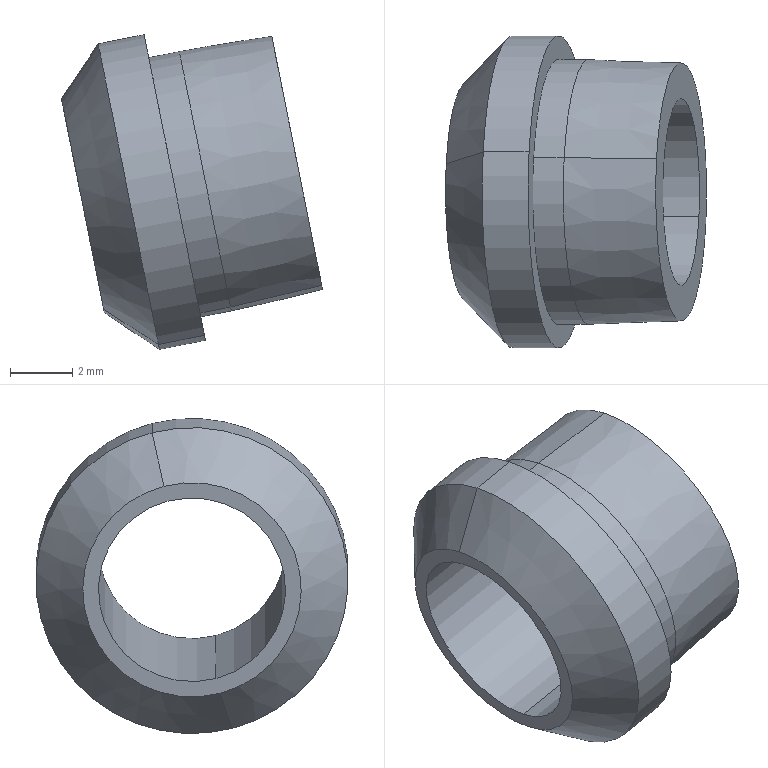Component | SolidWorks | 3-1 | 1 solid | 13 faces | box 8.37 x 10 x 10.1 mm | volume 229 mm3 | cylinder 6 | cone 4 | plane 3 | commonest cylinder face diameters 8.5 x2 10 x2 6 x2
build123d program:
from build123d import *

# Parameters (mm, degrees)
CHAMFER1_SIZE = 1.5


with BuildPart() as part:
    # Sketch1 → Revolve1 (revolve)
    with BuildSketch(Plane(origin=(0, 0, 0), x_dir=(1, 0, 0), z_dir=(0, 1, 0))):
        Polygon((0, 4.145), (3, 4.25), (4, 4.25), (4, 5), (7, 5), (7, 3), (0, 3), align=None)
    revolve(axis=Axis((7, 0, 0), (-1, 0, 0)))

    # Chamfer1
    chamfer1_edges = [part.edges().sort_by_distance(p)[0] for p in [
        (7, 0, 5),
    ]]
    chamfer(chamfer1_edges, length=CHAMFER1_SIZE)


solid = part.part

# Placed as in the assembly
solid = solid.moved(Location((91.677, -319.2, 18.375), (-89.807, -0.03862, 168.666)))
STEP:
#1=COLOUR_RGB('',0.7922,0.8196,0.9333);
#2=FILL_AREA_STYLE_COLOUR('',#1);
#3=FILL_AREA_STYLE('',(#2));
#4=SURFACE_STYLE_FILL_AREA(#3);
#5=SURFACE_SIDE_STYLE('',(#4));
#6=SURFACE_STYLE_USAGE(.BOTH.,#5);
#7=PRESENTATION_STYLE_ASSIGNMENT((#6));
#8=CARTESIAN_POINT('',(3.313,-12.532,0.7999));
#9=VERTEX_POINT('',#8);
#10=CARTESIAN_POINT('',(3.365,-12.602,0.5387));
#11=VERTEX_POINT('',#10);
#12=CARTESIAN_POINT('',(3.339,-12.567,0.6693));
#13=DIRECTION('',(-0.9805,-0.,-0.1965));
#14=DIRECTION('',(-0.19,0.2563,0.9478));
#15=AXIS2_PLACEMENT_3D('',#12,#13,#14);
#16=CIRCLE('',#15,0.1378);
#17=EDGE_CURVE('',#9,#11,#16,.T.);
#18=ORIENTED_EDGE('',*,*,#17,.F.);
#19=CARTESIAN_POINT('',(3.36,-12.516,0.8674));
#20=VERTEX_POINT('',#19);
#21=CARTESIAN_POINT('',(3.313,-12.532,0.7999));
#22=DIRECTION('',(0.559,0.1812,0.8091));
#23=VECTOR('',#22,39.37);
#24=LINE('',#21,#23);
#25=EDGE_CURVE('',#9,#20,#24,.T.);
#26=ORIENTED_EDGE('',*,*,#25,.T.);
#27=CARTESIAN_POINT('',(3.434,-12.617,0.4943));
#28=VERTEX_POINT('',#27);
#29=CARTESIAN_POINT('',(3.397,-12.567,0.6809));
#30=DIRECTION('',(0.9805,0.,0.1965));
#31=DIRECTION('',(-0.19,0.2563,0.9478));
#32=AXIS2_PLACEMENT_3D('',#29,#30,#31);
#33=CIRCLE('',#32,0.1969);
#34=EDGE_CURVE('',#28,#20,#33,.T.);
#35=ORIENTED_EDGE('',*,*,#34,.F.);
#36=CARTESIAN_POINT('',(3.365,-12.602,0.5387));
#37=DIRECTION('',(0.8276,-0.1812,-0.5312));
#38=VECTOR('',#37,39.37);
#39=LINE('',#36,#38);
#40=EDGE_CURVE('',#11,#28,#39,.T.);
#41=ORIENTED_EDGE('',*,*,#40,.F.);
#42=EDGE_LOOP('',(#18,#26,#35,#41));
#43=FACE_OUTER_BOUND('',#42,.T.);
#44=CARTESIAN_POINT('',(3.339,-12.567,0.6693));
#45=DIRECTION('',(0.9805,0.,0.1965));
#46=DIRECTION('',(0.19,-0.2563,-0.9478));
#47=AXIS2_PLACEMENT_3D('',#44,#45,#46);
#48=CONICAL_SURFACE('',#47,0.1378,0.7854);
#49=ADVANCED_FACE('',(#43),#48,.T.);
#50=CARTESIAN_POINT('',(3.578,-12.525,0.8781));
#51=VERTEX_POINT('',#50);
#52=CARTESIAN_POINT('',(3.64,-12.609,0.5687));
#53=VERTEX_POINT('',#52);
#54=CARTESIAN_POINT('',(3.609,-12.567,0.7234));
#55=DIRECTION('',(-0.9805,-0.,-0.1965));
#56=DIRECTION('',(-0.19,0.2563,0.9478));
#57=AXIS2_PLACEMENT_3D('',#54,#55,#56);
#58=CIRCLE('',#57,0.1632);
#59=EDGE_CURVE('',#51,#53,#58,.T.);
#60=ORIENTED_EDGE('',*,*,#59,.T.);
#61=CARTESIAN_POINT('',(3.525,-12.61,0.5416));
#62=VERTEX_POINT('',#61);
#63=CARTESIAN_POINT('',(3.525,-12.61,0.5416));
#64=DIRECTION('',(-0.9733,-0.008944,-0.2295));
#65=VECTOR('',#64,39.37);
#66=LINE('',#63,#65);
#67=EDGE_CURVE('',#53,#62,#66,.T.);
#68=ORIENTED_EDGE('',*,*,#67,.T.);
#69=CARTESIAN_POINT('',(3.462,-12.524,0.8588));
#70=VERTEX_POINT('',#69);
#71=CARTESIAN_POINT('',(3.494,-12.567,0.7002));
#72=DIRECTION('',(-0.9805,-0.,-0.1965));
#73=DIRECTION('',(-0.19,0.2563,0.9478));
#74=AXIS2_PLACEMENT_3D('',#71,#72,#73);
#75=CIRCLE('',#74,0.1673);
#76=EDGE_CURVE('',#70,#62,#75,.T.);
#77=ORIENTED_EDGE('',*,*,#76,.F.);
#78=CARTESIAN_POINT('',(3.462,-12.524,0.8588));
#79=DIRECTION('',(-0.9865,0.008944,-0.1633));
#80=VECTOR('',#79,39.37);
#81=LINE('',#78,#80);
#82=EDGE_CURVE('',#51,#70,#81,.T.);
#83=ORIENTED_EDGE('',*,*,#82,.F.);
#84=EDGE_LOOP('',(#60,#68,#77,#83));
#85=FACE_OUTER_BOUND('',#84,.T.);
#86=CARTESIAN_POINT('',(3.494,-12.567,0.7002));
#87=DIRECTION('',(-0.9805,-0.,-0.1965));
#88=DIRECTION('',(-0.19,0.2563,0.9478));
#89=AXIS2_PLACEMENT_3D('',#86,#87,#88);
#90=CONICAL_SURFACE('',#89,0.1673,0.03491);
#91=ADVANCED_FACE('',(#85),#90,.T.);
#92=ORIENTED_EDGE('',*,*,#76,.T.);
#93=CARTESIAN_POINT('',(3.487,-12.61,0.5339));
#94=VERTEX_POINT('',#93);
#95=CARTESIAN_POINT('',(3.371,-12.61,0.5107));
#96=DIRECTION('',(-0.9805,-0.,-0.1965));
#97=VECTOR('',#96,39.37);
#98=LINE('',#95,#97);
#99=EDGE_CURVE('',#62,#94,#98,.T.);
#100=ORIENTED_EDGE('',*,*,#99,.T.);
#101=CARTESIAN_POINT('',(3.423,-12.524,0.851));
#102=VERTEX_POINT('',#101);
#103=CARTESIAN_POINT('',(3.455,-12.567,0.6925));
#104=DIRECTION('',(-0.9805,-0.,-0.1965));
#105=DIRECTION('',(-0.19,0.2563,0.9478));
#106=AXIS2_PLACEMENT_3D('',#103,#104,#105);
#107=CIRCLE('',#106,0.1673);
#108=EDGE_CURVE('',#102,#94,#107,.T.);
#109=ORIENTED_EDGE('',*,*,#108,.F.);
#110=CARTESIAN_POINT('',(3.307,-12.524,0.8278));
#111=DIRECTION('',(-0.9805,-0.,-0.1965));
#112=VECTOR('',#111,39.37);
#113=LINE('',#110,#112);
#114=EDGE_CURVE('',#70,#102,#113,.T.);
#115=ORIENTED_EDGE('',*,*,#114,.F.);
#116=EDGE_LOOP('',(#92,#100,#109,#115));
#117=FACE_OUTER_BOUND('',#116,.T.);
#118=CARTESIAN_POINT('',(3.339,-12.567,0.6693));
#119=DIRECTION('',(-0.9805,-0.,-0.1965));
#120=DIRECTION('',(-0.19,0.2563,0.9478));
#121=AXIS2_PLACEMENT_3D('',#118,#119,#120);
#122=CYLINDRICAL_SURFACE('',#121,0.1673);
#123=ADVANCED_FACE('',(#117),#122,.T.);
#124=CARTESIAN_POINT('',(3.418,-12.516,0.879));
#125=VERTEX_POINT('',#124);
#126=CARTESIAN_POINT('',(3.492,-12.617,0.5059));
#127=VERTEX_POINT('',#126);
#128=CARTESIAN_POINT('',(3.455,-12.567,0.6925));
#129=DIRECTION('',(-0.9805,-0.,-0.1965));
#130=DIRECTION('',(-0.19,0.2563,0.9478));
#131=AXIS2_PLACEMENT_3D('',#128,#129,#130);
#132=CIRCLE('',#131,0.1969);
#133=EDGE_CURVE('',#125,#127,#132,.T.);
#134=ORIENTED_EDGE('',*,*,#133,.T.);
#135=CARTESIAN_POINT('',(3.376,-12.617,0.4827));
#136=DIRECTION('',(-0.9805,-0.,-0.1965));
#137=VECTOR('',#136,39.37);
#138=LINE('',#135,#137);
#139=EDGE_CURVE('',#127,#28,#138,.T.);
#140=ORIENTED_EDGE('',*,*,#139,.T.);
#141=ORIENTED_EDGE('',*,*,#34,.T.);
#142=CARTESIAN_POINT('',(3.302,-12.516,0.8558));
#143=DIRECTION('',(-0.9805,-0.,-0.1965));
#144=VECTOR('',#143,39.37);
#145=LINE('',#142,#144);
#146=EDGE_CURVE('',#125,#20,#145,.T.);
#147=ORIENTED_EDGE('',*,*,#146,.F.);
#148=EDGE_LOOP('',(#134,#140,#141,#147));
#149=FACE_OUTER_BOUND('',#148,.T.);
#150=CARTESIAN_POINT('',(3.339,-12.567,0.6693));
#151=DIRECTION('',(-0.9805,-0.,-0.1965));
#152=DIRECTION('',(-0.19,0.2563,0.9478));
#153=AXIS2_PLACEMENT_3D('',#150,#151,#152);
#154=CYLINDRICAL_SURFACE('',#153,0.1969);
#155=ADVANCED_FACE('',(#149),#154,.T.);
#156=CARTESIAN_POINT('',(3.632,-12.597,0.6115));
#157=VERTEX_POINT('',#156);
#158=CARTESIAN_POINT('',(3.587,-12.537,0.8354));
#159=VERTEX_POINT('',#158);
#160=CARTESIAN_POINT('',(3.609,-12.567,0.7234));
#161=DIRECTION('',(-0.9805,-0.,-0.1965));
#162=DIRECTION('',(-0.19,0.2563,0.9478));
#163=AXIS2_PLACEMENT_3D('',#160,#161,#162);
#164=CIRCLE('',#163,0.1181);
#165=EDGE_CURVE('',#157,#159,#164,.T.);
#166=ORIENTED_EDGE('',*,*,#165,.F.);
#167=CARTESIAN_POINT('',(3.362,-12.597,0.5573));
#168=VERTEX_POINT('',#167);
#169=CARTESIAN_POINT('',(3.362,-12.597,0.5573));
#170=DIRECTION('',(-0.9805,-0.,-0.1965));
#171=VECTOR('',#170,39.37);
#172=LINE('',#169,#171);
#173=EDGE_CURVE('',#157,#168,#172,.T.);
#174=ORIENTED_EDGE('',*,*,#173,.T.);
#175=CARTESIAN_POINT('',(3.317,-12.537,0.7812));
#176=VERTEX_POINT('',#175);
#177=CARTESIAN_POINT('',(3.339,-12.567,0.6693));
#178=DIRECTION('',(-0.9805,-0.,-0.1965));
#179=DIRECTION('',(-0.19,0.2563,0.9478));
#180=AXIS2_PLACEMENT_3D('',#177,#178,#179);
#181=CIRCLE('',#180,0.1181);
#182=EDGE_CURVE('',#168,#176,#181,.T.);
#183=ORIENTED_EDGE('',*,*,#182,.T.);
#184=CARTESIAN_POINT('',(3.317,-12.537,0.7812));
#185=DIRECTION('',(-0.9805,-0.,-0.1965));
#186=VECTOR('',#185,39.37);
#187=LINE('',#184,#186);
#188=EDGE_CURVE('',#159,#176,#187,.T.);
#189=ORIENTED_EDGE('',*,*,#188,.F.);
#190=EDGE_LOOP('',(#166,#174,#183,#189));
#191=FACE_OUTER_BOUND('',#190,.T.);
#192=CARTESIAN_POINT('',(3.339,-12.567,0.6693));
#193=DIRECTION('',(-0.9805,-0.,-0.1965));
#194=DIRECTION('',(-0.19,0.2563,0.9478));
#195=AXIS2_PLACEMENT_3D('',#192,#193,#194);
#196=CYLINDRICAL_SURFACE('',#195,0.1181);
#197=ADVANCED_FACE('',(#191),#196,.F.);
#198=CARTESIAN_POINT('',(3.609,-12.567,0.7234));
#199=DIRECTION('',(-0.9805,-0.,-0.1965));
#200=DIRECTION('',(-0.19,0.2563,0.9478));
#201=AXIS2_PLACEMENT_3D('',#198,#199,#200);
#202=CIRCLE('',#201,0.1181);
#203=EDGE_CURVE('',#159,#157,#202,.T.);
#204=ORIENTED_EDGE('',*,*,#203,.T.);
#205=ORIENTED_EDGE('',*,*,#165,.T.);
#206=EDGE_LOOP('',(#204,#205));
#207=FACE_BOUND('',#206,.T.);
#208=ORIENTED_EDGE('',*,*,#59,.F.);
#209=CARTESIAN_POINT('',(3.609,-12.567,0.7234));
#210=DIRECTION('',(-0.9805,-0.,-0.1965));
#211=DIRECTION('',(-0.19,0.2563,0.9478));
#212=AXIS2_PLACEMENT_3D('',#209,#210,#211);
#213=CIRCLE('',#212,0.1632);
#214=EDGE_CURVE('',#53,#51,#213,.T.);
#215=ORIENTED_EDGE('',*,*,#214,.F.);
#216=EDGE_LOOP('',(#208,#215));
#217=FACE_OUTER_BOUND('',#216,.T.);
#218=CARTESIAN_POINT('',(3.578,-12.525,0.8781));
#219=DIRECTION('',(0.9805,0.,0.1965));
#220=DIRECTION('',(0.19,-0.2563,-0.9478));
#221=AXIS2_PLACEMENT_3D('',#218,#219,#220);
#222=PLANE('',#221);
#223=ADVANCED_FACE('',(#207,#217),#222,.T.);
#224=ORIENTED_EDGE('',*,*,#173,.F.);
#225=ORIENTED_EDGE('',*,*,#203,.F.);
#226=ORIENTED_EDGE('',*,*,#188,.T.);
#227=CARTESIAN_POINT('',(3.339,-12.567,0.6693));
#228=DIRECTION('',(-0.9805,-0.,-0.1965));
#229=DIRECTION('',(-0.19,0.2563,0.9478));
#230=AXIS2_PLACEMENT_3D('',#227,#228,#229);
#231=CIRCLE('',#230,0.1181);
#232=EDGE_CURVE('',#176,#168,#231,.T.);
#233=ORIENTED_EDGE('',*,*,#232,.T.);
#234=EDGE_LOOP('',(#224,#225,#226,#233));
#235=FACE_OUTER_BOUND('',#234,.T.);
#236=CARTESIAN_POINT('',(3.339,-12.567,0.6693));
#237=DIRECTION('',(-0.9805,-0.,-0.1965));
#238=DIRECTION('',(-0.19,0.2563,0.9478));
#239=AXIS2_PLACEMENT_3D('',#236,#237,#238);
#240=CYLINDRICAL_SURFACE('',#239,0.1181);
#241=ADVANCED_FACE('',(#235),#240,.F.);
#242=CARTESIAN_POINT('',(3.339,-12.567,0.6693));
#243=DIRECTION('',(-0.9805,-0.,-0.1965));
#244=DIRECTION('',(-0.19,0.2563,0.9478));
#245=AXIS2_PLACEMENT_3D('',#242,#243,#244);
#246=CIRCLE('',#245,0.1378);
#247=EDGE_CURVE('',#11,#9,#246,.T.);
#248=ORIENTED_EDGE('',*,*,#247,.T.);
#249=ORIENTED_EDGE('',*,*,#17,.T.);
#250=EDGE_LOOP('',(#248,#249));
#251=FACE_OUTER_BOUND('',#250,.T.);
#252=ORIENTED_EDGE('',*,*,#232,.F.);
#253=ORIENTED_EDGE('',*,*,#182,.F.);
#254=EDGE_LOOP('',(#252,#253));
#255=FACE_BOUND('',#254,.T.);
#256=CARTESIAN_POINT('',(3.302,-12.516,0.8558));
#257=DIRECTION('',(-0.9805,-0.,-0.1965));
#258=DIRECTION('',(-0.19,0.2563,0.9478));
#259=AXIS2_PLACEMENT_3D('',#256,#257,#258);
#260=PLANE('',#259);
#261=ADVANCED_FACE('',(#251,#255),#260,.T.);
#262=ORIENTED_EDGE('',*,*,#139,.F.);
#263=CARTESIAN_POINT('',(3.455,-12.567,0.6925));
#264=DIRECTION('',(-0.9805,-0.,-0.1965));
#265=DIRECTION('',(-0.19,0.2563,0.9478));
#266=AXIS2_PLACEMENT_3D('',#263,#264,#265);
#267=CIRCLE('',#266,0.1969);
#268=EDGE_CURVE('',#127,#125,#267,.T.);
#269=ORIENTED_EDGE('',*,*,#268,.T.);
#270=ORIENTED_EDGE('',*,*,#146,.T.);
#271=CARTESIAN_POINT('',(3.397,-12.567,0.6809));
#272=DIRECTION('',(0.9805,0.,0.1965));
#273=DIRECTION('',(-0.19,0.2563,0.9478));
#274=AXIS2_PLACEMENT_3D('',#271,#272,#273);
#275=CIRCLE('',#274,0.1969);
#276=EDGE_CURVE('',#20,#28,#275,.T.);
#277=ORIENTED_EDGE('',*,*,#276,.T.);
#278=EDGE_LOOP('',(#262,#269,#270,#277));
#279=FACE_OUTER_BOUND('',#278,.T.);
#280=CARTESIAN_POINT('',(3.339,-12.567,0.6693));
#281=DIRECTION('',(-0.9805,-0.,-0.1965));
#282=DIRECTION('',(-0.19,0.2563,0.9478));
#283=AXIS2_PLACEMENT_3D('',#280,#281,#282);
#284=CYLINDRICAL_SURFACE('',#283,0.1969);
#285=ADVANCED_FACE('',(#279),#284,.T.);
#286=ORIENTED_EDGE('',*,*,#108,.T.);
#287=CARTESIAN_POINT('',(3.455,-12.567,0.6925));
#288=DIRECTION('',(-0.9805,-0.,-0.1965));
#289=DIRECTION('',(-0.19,0.2563,0.9478));
#290=AXIS2_PLACEMENT_3D('',#287,#288,#289);
#291=CIRCLE('',#290,0.1673);
#292=EDGE_CURVE('',#94,#102,#291,.T.);
#293=ORIENTED_EDGE('',*,*,#292,.T.);
#294=EDGE_LOOP('',(#286,#293));
#295=FACE_BOUND('',#294,.T.);
#296=ORIENTED_EDGE('',*,*,#133,.F.);
#297=ORIENTED_EDGE('',*,*,#268,.F.);
#298=EDGE_LOOP('',(#296,#297));
#299=FACE_OUTER_BOUND('',#298,.T.);
#300=CARTESIAN_POINT('',(3.423,-12.524,0.851));
#301=DIRECTION('',(0.9805,0.,0.1965));
#302=DIRECTION('',(0.19,-0.2563,-0.9478));
#303=AXIS2_PLACEMENT_3D('',#300,#301,#302);
#304=PLANE('',#303);
#305=ADVANCED_FACE('',(#295,#299),#304,.T.);
#306=ORIENTED_EDGE('',*,*,#99,.F.);
#307=CARTESIAN_POINT('',(3.494,-12.567,0.7002));
#308=DIRECTION('',(-0.9805,-0.,-0.1965));
#309=DIRECTION('',(-0.19,0.2563,0.9478));
#310=AXIS2_PLACEMENT_3D('',#307,#308,#309);
#311=CIRCLE('',#310,0.1673);
#312=EDGE_CURVE('',#62,#70,#311,.T.);
#313=ORIENTED_EDGE('',*,*,#312,.T.);
#314=ORIENTED_EDGE('',*,*,#114,.T.);
#315=ORIENTED_EDGE('',*,*,#292,.F.);
#316=EDGE_LOOP('',(#306,#313,#314,#315));
#317=FACE_OUTER_BOUND('',#316,.T.);
#318=CARTESIAN_POINT('',(3.339,-12.567,0.6693));
#319=DIRECTION('',(-0.9805,-0.,-0.1965));
#320=DIRECTION('',(-0.19,0.2563,0.9478));
#321=AXIS2_PLACEMENT_3D('',#318,#319,#320);
#322=CYLINDRICAL_SURFACE('',#321,0.1673);
#323=ADVANCED_FACE('',(#317),#322,.T.);
#324=ORIENTED_EDGE('',*,*,#67,.F.);
#325=ORIENTED_EDGE('',*,*,#214,.T.);
#326=ORIENTED_EDGE('',*,*,#82,.T.);
#327=ORIENTED_EDGE('',*,*,#312,.F.);
#328=EDGE_LOOP('',(#324,#325,#326,#327));
#329=FACE_OUTER_BOUND('',#328,.T.);
#330=CARTESIAN_POINT('',(3.494,-12.567,0.7002));
#331=DIRECTION('',(-0.9805,-0.,-0.1965));
#332=DIRECTION('',(-0.19,0.2563,0.9478));
#333=AXIS2_PLACEMENT_3D('',#330,#331,#332);
#334=CONICAL_SURFACE('',#333,0.1673,0.03491);
#335=ADVANCED_FACE('',(#329),#334,.T.);
#336=ORIENTED_EDGE('',*,*,#25,.F.);
#337=ORIENTED_EDGE('',*,*,#247,.F.);
#338=ORIENTED_EDGE('',*,*,#40,.T.);
#339=ORIENTED_EDGE('',*,*,#276,.F.);
#340=EDGE_LOOP('',(#336,#337,#338,#339));
#341=FACE_OUTER_BOUND('',#340,.T.);
#342=CARTESIAN_POINT('',(3.339,-12.567,0.6693));
#343=DIRECTION('',(0.9805,0.,0.1965));
#344=DIRECTION('',(0.19,-0.2563,-0.9478));
#345=AXIS2_PLACEMENT_3D('',#342,#343,#344);
#346=CONICAL_SURFACE('',#345,0.1378,0.7854);
#347=ADVANCED_FACE('',(#341),#346,.T.);
#348=CLOSED_SHELL('',(#49,#91,#123,#155,#197,#223,#241,#261,#285,#305,#323,#335,#347));
#349=MANIFOLD_SOLID_BREP('',#348);
#350=STYLED_ITEM('',(#7),#349);
#351=PRESENTATION_LAYER_ASSIGNMENT('','',(#350));
#352=(LENGTH_UNIT()NAMED_UNIT(*)SI_UNIT($,.METRE.));
#353=LENGTH_MEASURE_WITH_UNIT(LENGTH_MEASURE(0.0254),#352);
#354=DIMENSIONAL_EXPONENTS(1.,0.,0.,0.,0.,0.,0.);
#355=(CONVERSION_BASED_UNIT('',#353)LENGTH_UNIT()NAMED_UNIT(#354));
#356=UNCERTAINTY_MEASURE_WITH_UNIT(LENGTH_MEASURE(0.00001),#355,'','');
#357=(NAMED_UNIT(*)PLANE_ANGLE_UNIT()SI_UNIT($,.RADIAN.));
#358=(NAMED_UNIT(*)SI_UNIT($,.STERADIAN.)SOLID_ANGLE_UNIT());
#359=(GEOMETRIC_REPRESENTATION_CONTEXT(3)GLOBAL_UNCERTAINTY_ASSIGNED_CONTEXT((#356))GLOBAL_UNIT_ASSIGNED_CONTEXT((#355,#357,#358))REPRESENTATION_CONTEXT('',''));
#360=MECHANICAL_DESIGN_GEOMETRIC_PRESENTATION_REPRESENTATION('',(#350),#359);
#361=CARTESIAN_POINT('',(0.,0.,0.));
#362=DIRECTION('',(0.,0.,1.));
#363=DIRECTION('',(1.,0.,0.));
#364=AXIS2_PLACEMENT_3D('',#361,#362,#363);
#365=(LENGTH_UNIT()NAMED_UNIT(*)SI_UNIT($,.METRE.));
#366=LENGTH_MEASURE_WITH_UNIT(LENGTH_MEASURE(0.0254),#365);
#367=DIMENSIONAL_EXPONENTS(1.,0.,0.,0.,0.,0.,0.);
#368=(CONVERSION_BASED_UNIT('',#366)LENGTH_UNIT()NAMED_UNIT(#367));
#369=UNCERTAINTY_MEASURE_WITH_UNIT(LENGTH_MEASURE(0.00001),#368,'','');
#370=(NAMED_UNIT(*)PLANE_ANGLE_UNIT()SI_UNIT($,.RADIAN.));
#371=(NAMED_UNIT(*)SI_UNIT($,.STERADIAN.)SOLID_ANGLE_UNIT());
#372=(GEOMETRIC_REPRESENTATION_CONTEXT(3)GLOBAL_UNCERTAINTY_ASSIGNED_CONTEXT((#369))GLOBAL_UNIT_ASSIGNED_CONTEXT((#368,#370,#371))REPRESENTATION_CONTEXT('',''));
#373=ADVANCED_BREP_SHAPE_REPRESENTATION('',(#349,#364),#372);